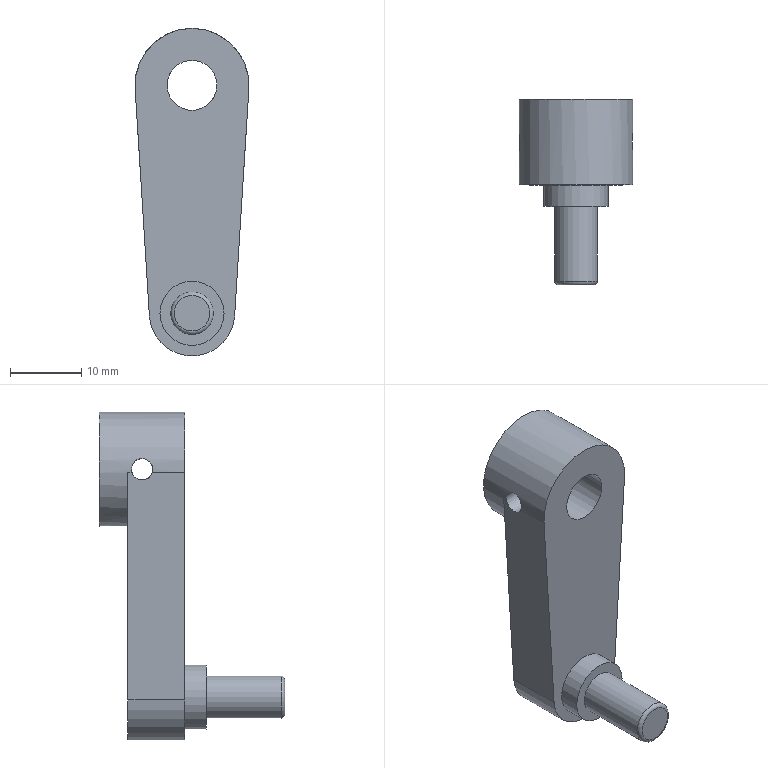Component | NX | CAM | 1 solid | 15 faces | volume 5627 mm3 | cylinder 7 | plane 7 | torus 1 | commonest cylinder face diameters 3 x2 16 x1 7 x1 12 x1 9 x1 6 x1